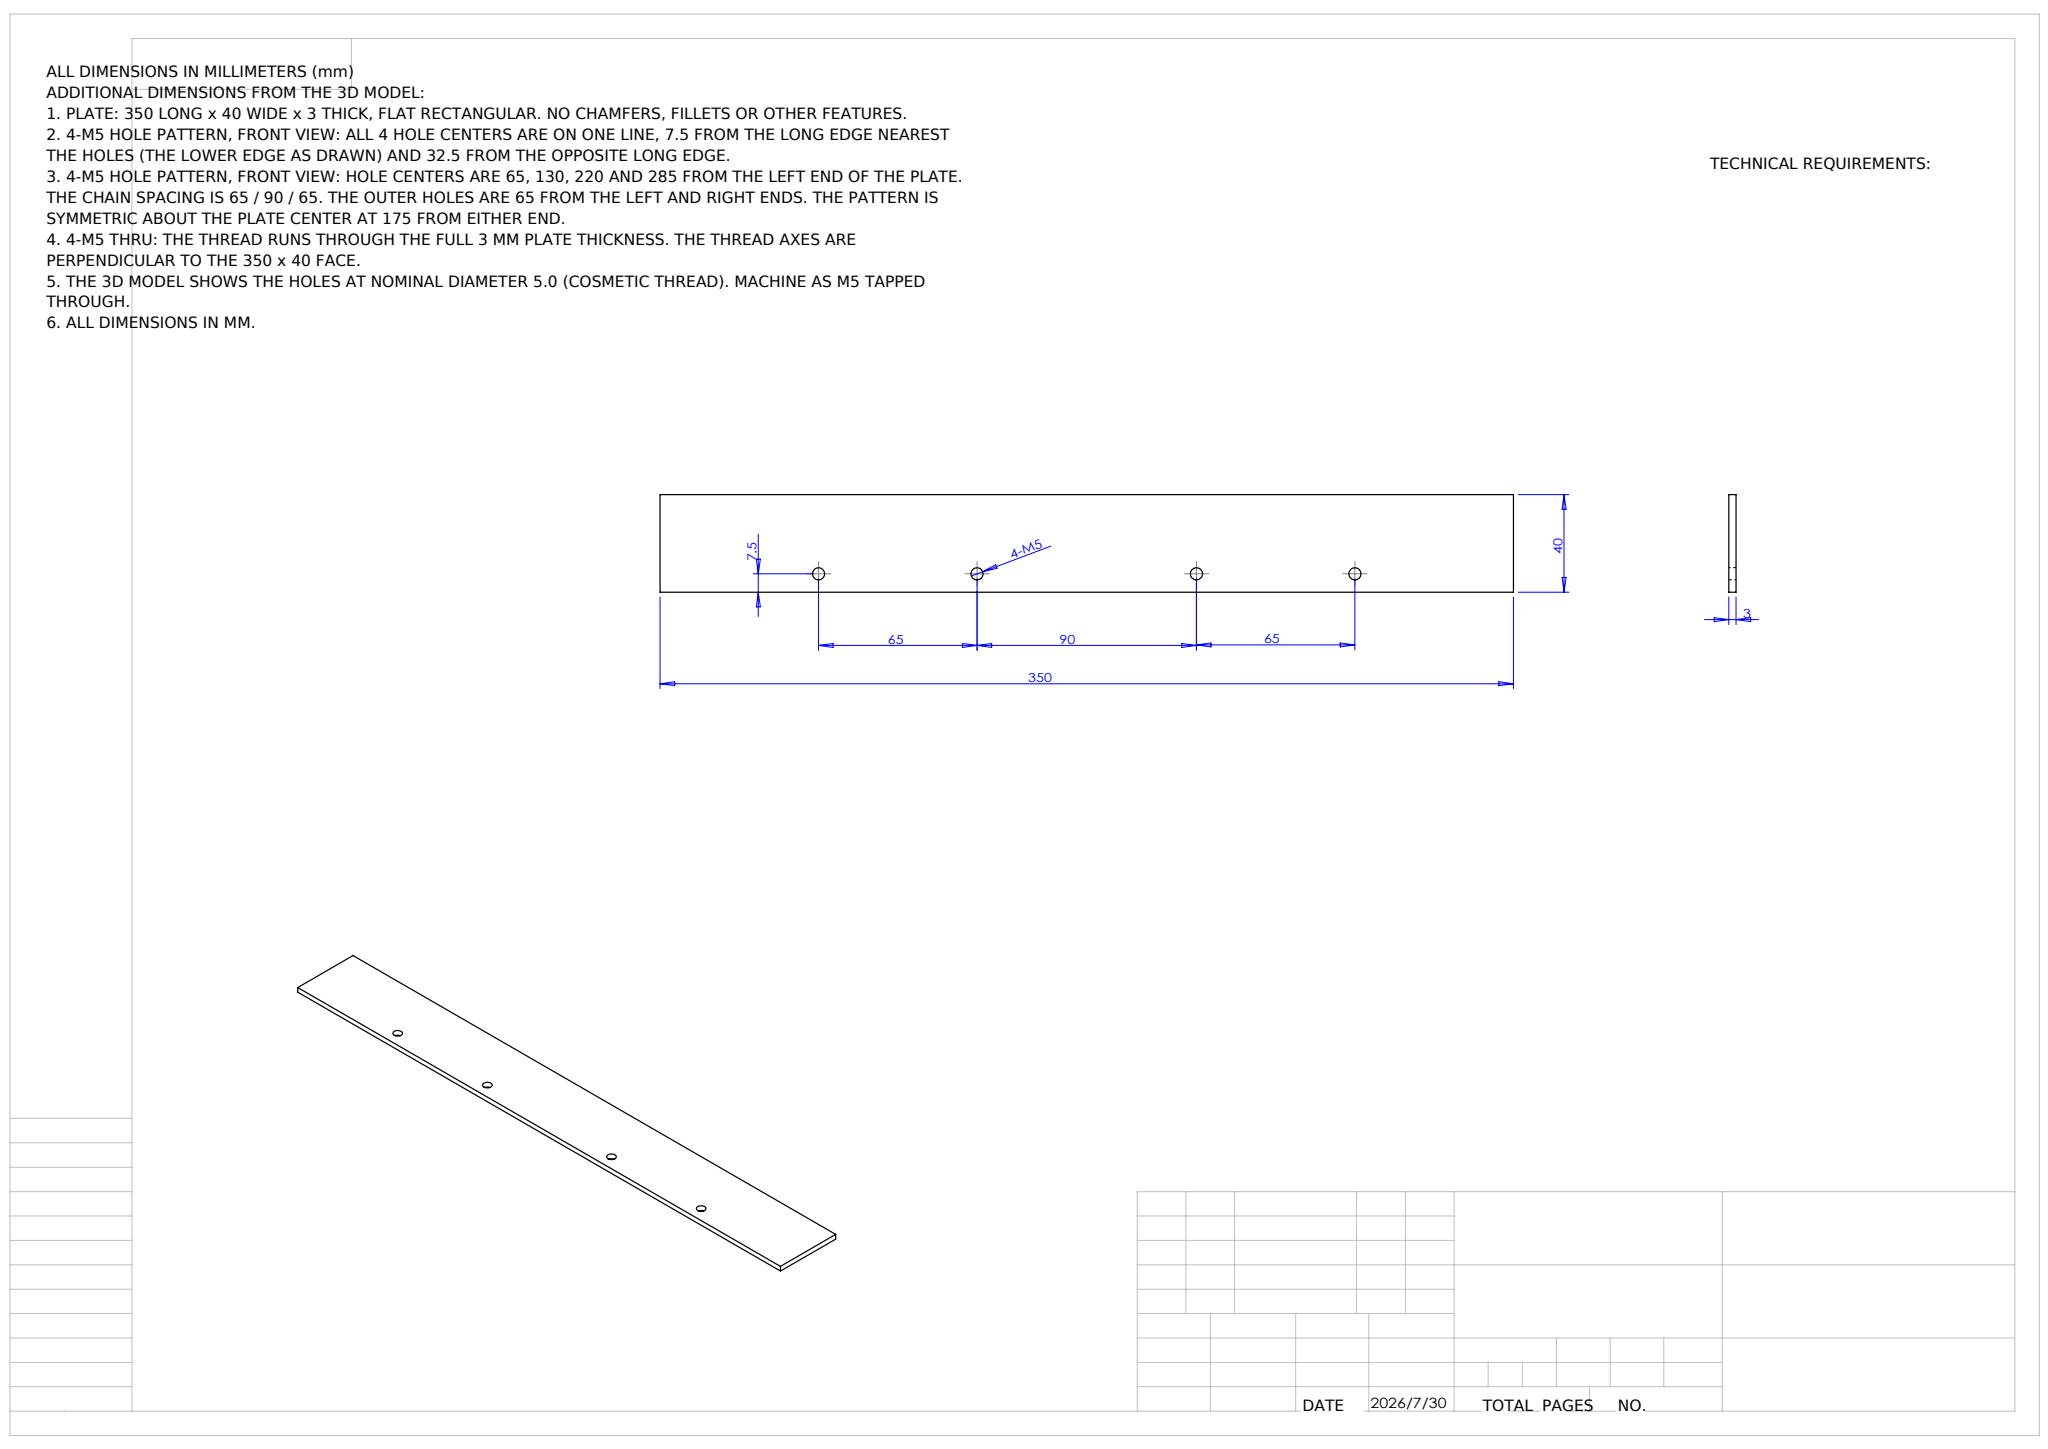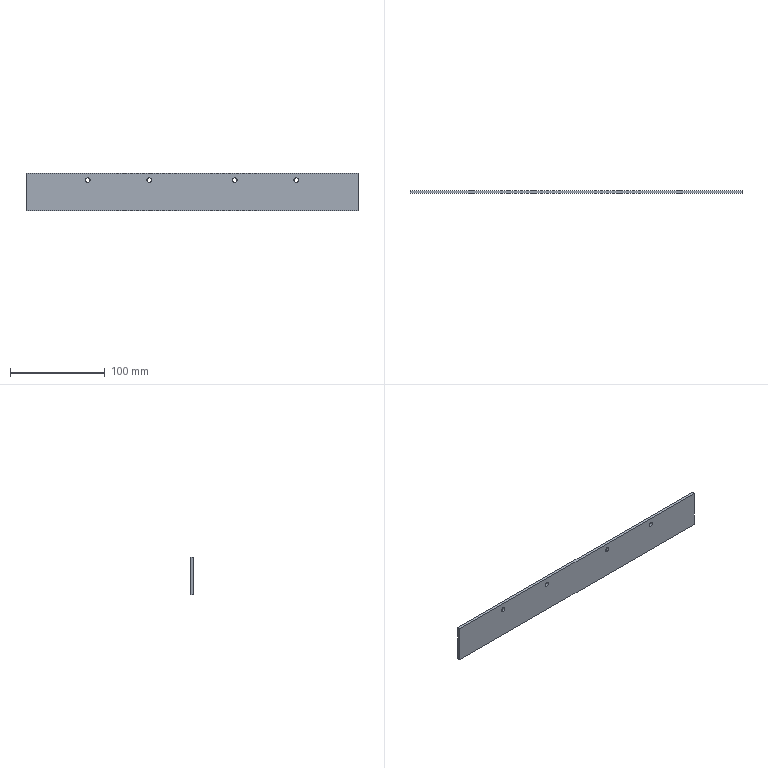Part | NX | mm | 1 solid | 14 faces | box 350 x 3 x 40 mm | volume 41764 mm3 | cylinder 8 | plane 6 | commonest cylinder face diameters 5 x8
STEP:
#1=COLOUR_RGB('',0.7529,0.7529,0.7529);
#2=FILL_AREA_STYLE_COLOUR('',#1);
#3=FILL_AREA_STYLE('',(#2));
#4=SURFACE_STYLE_FILL_AREA(#3);
#5=SURFACE_SIDE_STYLE('',(#4));
#6=SURFACE_STYLE_USAGE(.BOTH.,#5);
#7=PRESENTATION_STYLE_ASSIGNMENT((#6));
#8=CARTESIAN_POINT('',(23.046,0.,5.261));
#9=VERTEX_POINT('',#8);
#10=CARTESIAN_POINT('',(23.046,0.,10.261));
#11=VERTEX_POINT('',#10);
#12=CARTESIAN_POINT('',(23.046,0.,7.761));
#13=DIRECTION('',(0.,1.,0.));
#14=DIRECTION('',(0.,0.,1.));
#15=AXIS2_PLACEMENT_3D('',#12,#13,#14);
#16=CIRCLE('',#15,2.5);
#17=EDGE_CURVE('',#9,#11,#16,.T.);
#18=ORIENTED_EDGE('',*,*,#17,.F.);
#19=CARTESIAN_POINT('',(23.046,3.,5.261));
#20=VERTEX_POINT('',#19);
#21=CARTESIAN_POINT('',(23.046,0.,5.261));
#22=DIRECTION('',(0.,1.,0.));
#23=VECTOR('',#22,1000.);
#24=LINE('',#21,#23);
#25=EDGE_CURVE('',#9,#20,#24,.T.);
#26=ORIENTED_EDGE('',*,*,#25,.T.);
#27=CARTESIAN_POINT('',(23.046,3.,10.261));
#28=VERTEX_POINT('',#27);
#29=CARTESIAN_POINT('',(23.046,3.,7.761));
#30=DIRECTION('',(0.,1.,0.));
#31=DIRECTION('',(0.,0.,1.));
#32=AXIS2_PLACEMENT_3D('',#29,#30,#31);
#33=CIRCLE('',#32,2.5);
#34=EDGE_CURVE('',#20,#28,#33,.T.);
#35=ORIENTED_EDGE('',*,*,#34,.T.);
#36=CARTESIAN_POINT('',(23.046,0.,10.261));
#37=DIRECTION('',(0.,1.,0.));
#38=VECTOR('',#37,1000.);
#39=LINE('',#36,#38);
#40=EDGE_CURVE('',#11,#28,#39,.T.);
#41=ORIENTED_EDGE('',*,*,#40,.F.);
#42=EDGE_LOOP('',(#18,#26,#35,#41));
#43=FACE_OUTER_BOUND('',#42,.T.);
#44=CARTESIAN_POINT('',(23.046,0.,7.761));
#45=DIRECTION('',(0.,1.,0.));
#46=DIRECTION('',(0.,0.,1.));
#47=AXIS2_PLACEMENT_3D('',#44,#45,#46);
#48=CYLINDRICAL_SURFACE('',#47,2.5);
#49=ADVANCED_FACE('',(#43),#48,.F.);
#50=CARTESIAN_POINT('',(-41.954,0.,5.261));
#51=VERTEX_POINT('',#50);
#52=CARTESIAN_POINT('',(-41.954,0.,10.261));
#53=VERTEX_POINT('',#52);
#54=CARTESIAN_POINT('',(-41.954,0.,7.761));
#55=DIRECTION('',(0.,1.,0.));
#56=DIRECTION('',(0.,0.,1.));
#57=AXIS2_PLACEMENT_3D('',#54,#55,#56);
#58=CIRCLE('',#57,2.5);
#59=EDGE_CURVE('',#51,#53,#58,.T.);
#60=ORIENTED_EDGE('',*,*,#59,.F.);
#61=CARTESIAN_POINT('',(-41.954,3.,5.261));
#62=VERTEX_POINT('',#61);
#63=CARTESIAN_POINT('',(-41.954,0.,5.261));
#64=DIRECTION('',(0.,1.,0.));
#65=VECTOR('',#64,1000.);
#66=LINE('',#63,#65);
#67=EDGE_CURVE('',#51,#62,#66,.T.);
#68=ORIENTED_EDGE('',*,*,#67,.T.);
#69=CARTESIAN_POINT('',(-41.954,3.,10.261));
#70=VERTEX_POINT('',#69);
#71=CARTESIAN_POINT('',(-41.954,3.,7.761));
#72=DIRECTION('',(0.,1.,0.));
#73=DIRECTION('',(0.,0.,1.));
#74=AXIS2_PLACEMENT_3D('',#71,#72,#73);
#75=CIRCLE('',#74,2.5);
#76=EDGE_CURVE('',#62,#70,#75,.T.);
#77=ORIENTED_EDGE('',*,*,#76,.T.);
#78=CARTESIAN_POINT('',(-41.954,0.,10.261));
#79=DIRECTION('',(0.,1.,0.));
#80=VECTOR('',#79,1000.);
#81=LINE('',#78,#80);
#82=EDGE_CURVE('',#53,#70,#81,.T.);
#83=ORIENTED_EDGE('',*,*,#82,.F.);
#84=EDGE_LOOP('',(#60,#68,#77,#83));
#85=FACE_OUTER_BOUND('',#84,.T.);
#86=CARTESIAN_POINT('',(-41.954,0.,7.761));
#87=DIRECTION('',(0.,1.,0.));
#88=DIRECTION('',(0.,0.,1.));
#89=AXIS2_PLACEMENT_3D('',#86,#87,#88);
#90=CYLINDRICAL_SURFACE('',#89,2.5);
#91=ADVANCED_FACE('',(#85),#90,.F.);
#92=CARTESIAN_POINT('',(-131.954,0.,5.261));
#93=VERTEX_POINT('',#92);
#94=CARTESIAN_POINT('',(-131.954,0.,10.261));
#95=VERTEX_POINT('',#94);
#96=CARTESIAN_POINT('',(-131.954,0.,7.761));
#97=DIRECTION('',(0.,1.,0.));
#98=DIRECTION('',(0.,0.,1.));
#99=AXIS2_PLACEMENT_3D('',#96,#97,#98);
#100=CIRCLE('',#99,2.5);
#101=EDGE_CURVE('',#93,#95,#100,.T.);
#102=ORIENTED_EDGE('',*,*,#101,.F.);
#103=CARTESIAN_POINT('',(-131.954,3.,5.261));
#104=VERTEX_POINT('',#103);
#105=CARTESIAN_POINT('',(-131.954,0.,5.261));
#106=DIRECTION('',(0.,1.,0.));
#107=VECTOR('',#106,1000.);
#108=LINE('',#105,#107);
#109=EDGE_CURVE('',#93,#104,#108,.T.);
#110=ORIENTED_EDGE('',*,*,#109,.T.);
#111=CARTESIAN_POINT('',(-131.954,3.,10.261));
#112=VERTEX_POINT('',#111);
#113=CARTESIAN_POINT('',(-131.954,3.,7.761));
#114=DIRECTION('',(0.,1.,0.));
#115=DIRECTION('',(0.,0.,1.));
#116=AXIS2_PLACEMENT_3D('',#113,#114,#115);
#117=CIRCLE('',#116,2.5);
#118=EDGE_CURVE('',#104,#112,#117,.T.);
#119=ORIENTED_EDGE('',*,*,#118,.T.);
#120=CARTESIAN_POINT('',(-131.954,0.,10.261));
#121=DIRECTION('',(0.,1.,0.));
#122=VECTOR('',#121,1000.);
#123=LINE('',#120,#122);
#124=EDGE_CURVE('',#95,#112,#123,.T.);
#125=ORIENTED_EDGE('',*,*,#124,.F.);
#126=EDGE_LOOP('',(#102,#110,#119,#125));
#127=FACE_OUTER_BOUND('',#126,.T.);
#128=CARTESIAN_POINT('',(-131.954,0.,7.761));
#129=DIRECTION('',(0.,1.,0.));
#130=DIRECTION('',(0.,0.,1.));
#131=AXIS2_PLACEMENT_3D('',#128,#129,#130);
#132=CYLINDRICAL_SURFACE('',#131,2.5);
#133=ADVANCED_FACE('',(#127),#132,.F.);
#134=CARTESIAN_POINT('',(-196.954,0.,5.261));
#135=VERTEX_POINT('',#134);
#136=CARTESIAN_POINT('',(-196.954,0.,10.261));
#137=VERTEX_POINT('',#136);
#138=CARTESIAN_POINT('',(-196.954,0.,7.761));
#139=DIRECTION('',(0.,1.,0.));
#140=DIRECTION('',(0.,0.,1.));
#141=AXIS2_PLACEMENT_3D('',#138,#139,#140);
#142=CIRCLE('',#141,2.5);
#143=EDGE_CURVE('',#135,#137,#142,.T.);
#144=ORIENTED_EDGE('',*,*,#143,.F.);
#145=CARTESIAN_POINT('',(-196.954,3.,5.261));
#146=VERTEX_POINT('',#145);
#147=CARTESIAN_POINT('',(-196.954,0.,5.261));
#148=DIRECTION('',(0.,1.,0.));
#149=VECTOR('',#148,1000.);
#150=LINE('',#147,#149);
#151=EDGE_CURVE('',#135,#146,#150,.T.);
#152=ORIENTED_EDGE('',*,*,#151,.T.);
#153=CARTESIAN_POINT('',(-196.954,3.,10.261));
#154=VERTEX_POINT('',#153);
#155=CARTESIAN_POINT('',(-196.954,3.,7.761));
#156=DIRECTION('',(0.,1.,0.));
#157=DIRECTION('',(0.,0.,1.));
#158=AXIS2_PLACEMENT_3D('',#155,#156,#157);
#159=CIRCLE('',#158,2.5);
#160=EDGE_CURVE('',#146,#154,#159,.T.);
#161=ORIENTED_EDGE('',*,*,#160,.T.);
#162=CARTESIAN_POINT('',(-196.954,0.,10.261));
#163=DIRECTION('',(0.,1.,0.));
#164=VECTOR('',#163,1000.);
#165=LINE('',#162,#164);
#166=EDGE_CURVE('',#137,#154,#165,.T.);
#167=ORIENTED_EDGE('',*,*,#166,.F.);
#168=EDGE_LOOP('',(#144,#152,#161,#167));
#169=FACE_OUTER_BOUND('',#168,.T.);
#170=CARTESIAN_POINT('',(-196.954,0.,7.761));
#171=DIRECTION('',(0.,1.,0.));
#172=DIRECTION('',(0.,0.,1.));
#173=AXIS2_PLACEMENT_3D('',#170,#171,#172);
#174=CYLINDRICAL_SURFACE('',#173,2.5);
#175=ADVANCED_FACE('',(#169),#174,.F.);
#176=CARTESIAN_POINT('',(-261.954,0.,-24.739));
#177=VERTEX_POINT('',#176);
#178=CARTESIAN_POINT('',(-261.954,0.,15.261));
#179=VERTEX_POINT('',#178);
#180=CARTESIAN_POINT('',(-261.954,0.,15.261));
#181=DIRECTION('',(0.,0.,1.));
#182=VECTOR('',#181,1000.);
#183=LINE('',#180,#182);
#184=EDGE_CURVE('',#177,#179,#183,.T.);
#185=ORIENTED_EDGE('',*,*,#184,.T.);
#186=CARTESIAN_POINT('',(-261.954,3.,15.261));
#187=VERTEX_POINT('',#186);
#188=CARTESIAN_POINT('',(-261.954,3.,15.261));
#189=DIRECTION('',(0.,-1.,0.));
#190=VECTOR('',#189,1000.);
#191=LINE('',#188,#190);
#192=EDGE_CURVE('',#187,#179,#191,.T.);
#193=ORIENTED_EDGE('',*,*,#192,.F.);
#194=CARTESIAN_POINT('',(-261.954,3.,-24.739));
#195=VERTEX_POINT('',#194);
#196=CARTESIAN_POINT('',(-261.954,3.,15.261));
#197=DIRECTION('',(0.,0.,1.));
#198=VECTOR('',#197,1000.);
#199=LINE('',#196,#198);
#200=EDGE_CURVE('',#195,#187,#199,.T.);
#201=ORIENTED_EDGE('',*,*,#200,.F.);
#202=CARTESIAN_POINT('',(-261.954,3.,-24.739));
#203=DIRECTION('',(0.,-1.,0.));
#204=VECTOR('',#203,1000.);
#205=LINE('',#202,#204);
#206=EDGE_CURVE('',#195,#177,#205,.T.);
#207=ORIENTED_EDGE('',*,*,#206,.T.);
#208=EDGE_LOOP('',(#185,#193,#201,#207));
#209=FACE_OUTER_BOUND('',#208,.T.);
#210=CARTESIAN_POINT('',(-261.954,3.,15.261));
#211=DIRECTION('',(1.,0.,0.));
#212=DIRECTION('',(0.,0.,-1.));
#213=AXIS2_PLACEMENT_3D('',#210,#211,#212);
#214=PLANE('',#213);
#215=ADVANCED_FACE('',(#209),#214,.F.);
#216=CARTESIAN_POINT('',(88.046,0.,15.261));
#217=VERTEX_POINT('',#216);
#218=CARTESIAN_POINT('',(-261.954,0.,15.261));
#219=DIRECTION('',(1.,0.,0.));
#220=VECTOR('',#219,1000.);
#221=LINE('',#218,#220);
#222=EDGE_CURVE('',#179,#217,#221,.T.);
#223=ORIENTED_EDGE('',*,*,#222,.T.);
#224=CARTESIAN_POINT('',(88.046,3.,15.261));
#225=VERTEX_POINT('',#224);
#226=CARTESIAN_POINT('',(88.046,3.,15.261));
#227=DIRECTION('',(0.,-1.,0.));
#228=VECTOR('',#227,1000.);
#229=LINE('',#226,#228);
#230=EDGE_CURVE('',#225,#217,#229,.T.);
#231=ORIENTED_EDGE('',*,*,#230,.F.);
#232=CARTESIAN_POINT('',(-261.954,3.,15.261));
#233=DIRECTION('',(1.,0.,0.));
#234=VECTOR('',#233,1000.);
#235=LINE('',#232,#234);
#236=EDGE_CURVE('',#187,#225,#235,.T.);
#237=ORIENTED_EDGE('',*,*,#236,.F.);
#238=ORIENTED_EDGE('',*,*,#192,.T.);
#239=EDGE_LOOP('',(#223,#231,#237,#238));
#240=FACE_OUTER_BOUND('',#239,.T.);
#241=CARTESIAN_POINT('',(-261.954,3.,15.261));
#242=DIRECTION('',(0.,0.,-1.));
#243=DIRECTION('',(-1.,0.,0.));
#244=AXIS2_PLACEMENT_3D('',#241,#242,#243);
#245=PLANE('',#244);
#246=ADVANCED_FACE('',(#240),#245,.F.);
#247=CARTESIAN_POINT('',(88.046,0.,-24.739));
#248=VERTEX_POINT('',#247);
#249=CARTESIAN_POINT('',(88.046,0.,15.261));
#250=DIRECTION('',(0.,0.,-1.));
#251=VECTOR('',#250,1000.);
#252=LINE('',#249,#251);
#253=EDGE_CURVE('',#217,#248,#252,.T.);
#254=ORIENTED_EDGE('',*,*,#253,.T.);
#255=CARTESIAN_POINT('',(88.046,3.,-24.739));
#256=VERTEX_POINT('',#255);
#257=CARTESIAN_POINT('',(88.046,3.,-24.739));
#258=DIRECTION('',(0.,-1.,0.));
#259=VECTOR('',#258,1000.);
#260=LINE('',#257,#259);
#261=EDGE_CURVE('',#256,#248,#260,.T.);
#262=ORIENTED_EDGE('',*,*,#261,.F.);
#263=CARTESIAN_POINT('',(88.046,3.,15.261));
#264=DIRECTION('',(0.,0.,-1.));
#265=VECTOR('',#264,1000.);
#266=LINE('',#263,#265);
#267=EDGE_CURVE('',#225,#256,#266,.T.);
#268=ORIENTED_EDGE('',*,*,#267,.F.);
#269=ORIENTED_EDGE('',*,*,#230,.T.);
#270=EDGE_LOOP('',(#254,#262,#268,#269));
#271=FACE_OUTER_BOUND('',#270,.T.);
#272=CARTESIAN_POINT('',(88.046,3.,15.261));
#273=DIRECTION('',(-1.,0.,0.));
#274=DIRECTION('',(0.,0.,1.));
#275=AXIS2_PLACEMENT_3D('',#272,#273,#274);
#276=PLANE('',#275);
#277=ADVANCED_FACE('',(#271),#276,.F.);
#278=CARTESIAN_POINT('',(-261.954,0.,-24.739));
#279=DIRECTION('',(-1.,0.,0.));
#280=VECTOR('',#279,1000.);
#281=LINE('',#278,#280);
#282=EDGE_CURVE('',#248,#177,#281,.T.);
#283=ORIENTED_EDGE('',*,*,#282,.T.);
#284=ORIENTED_EDGE('',*,*,#206,.F.);
#285=CARTESIAN_POINT('',(-261.954,3.,-24.739));
#286=DIRECTION('',(-1.,0.,0.));
#287=VECTOR('',#286,1000.);
#288=LINE('',#285,#287);
#289=EDGE_CURVE('',#256,#195,#288,.T.);
#290=ORIENTED_EDGE('',*,*,#289,.F.);
#291=ORIENTED_EDGE('',*,*,#261,.T.);
#292=EDGE_LOOP('',(#283,#284,#290,#291));
#293=FACE_OUTER_BOUND('',#292,.T.);
#294=CARTESIAN_POINT('',(-261.954,3.,-24.739));
#295=DIRECTION('',(0.,0.,1.));
#296=DIRECTION('',(1.,0.,0.));
#297=AXIS2_PLACEMENT_3D('',#294,#295,#296);
#298=PLANE('',#297);
#299=ADVANCED_FACE('',(#293),#298,.F.);
#300=CARTESIAN_POINT('',(23.046,3.,7.761));
#301=DIRECTION('',(0.,1.,0.));
#302=DIRECTION('',(0.,0.,1.));
#303=AXIS2_PLACEMENT_3D('',#300,#301,#302);
#304=CIRCLE('',#303,2.5);
#305=EDGE_CURVE('',#28,#20,#304,.T.);
#306=ORIENTED_EDGE('',*,*,#305,.F.);
#307=ORIENTED_EDGE('',*,*,#34,.F.);
#308=EDGE_LOOP('',(#306,#307));
#309=FACE_BOUND('',#308,.T.);
#310=CARTESIAN_POINT('',(-41.954,3.,7.761));
#311=DIRECTION('',(0.,1.,0.));
#312=DIRECTION('',(0.,0.,1.));
#313=AXIS2_PLACEMENT_3D('',#310,#311,#312);
#314=CIRCLE('',#313,2.5);
#315=EDGE_CURVE('',#70,#62,#314,.T.);
#316=ORIENTED_EDGE('',*,*,#315,.F.);
#317=ORIENTED_EDGE('',*,*,#76,.F.);
#318=EDGE_LOOP('',(#316,#317));
#319=FACE_BOUND('',#318,.T.);
#320=CARTESIAN_POINT('',(-131.954,3.,7.761));
#321=DIRECTION('',(0.,1.,0.));
#322=DIRECTION('',(0.,0.,1.));
#323=AXIS2_PLACEMENT_3D('',#320,#321,#322);
#324=CIRCLE('',#323,2.5);
#325=EDGE_CURVE('',#112,#104,#324,.T.);
#326=ORIENTED_EDGE('',*,*,#325,.F.);
#327=ORIENTED_EDGE('',*,*,#118,.F.);
#328=EDGE_LOOP('',(#326,#327));
#329=FACE_BOUND('',#328,.T.);
#330=CARTESIAN_POINT('',(-196.954,3.,7.761));
#331=DIRECTION('',(0.,1.,0.));
#332=DIRECTION('',(0.,0.,1.));
#333=AXIS2_PLACEMENT_3D('',#330,#331,#332);
#334=CIRCLE('',#333,2.5);
#335=EDGE_CURVE('',#154,#146,#334,.T.);
#336=ORIENTED_EDGE('',*,*,#335,.F.);
#337=ORIENTED_EDGE('',*,*,#160,.F.);
#338=EDGE_LOOP('',(#336,#337));
#339=FACE_BOUND('',#338,.T.);
#340=ORIENTED_EDGE('',*,*,#200,.T.);
#341=ORIENTED_EDGE('',*,*,#236,.T.);
#342=ORIENTED_EDGE('',*,*,#267,.T.);
#343=ORIENTED_EDGE('',*,*,#289,.T.);
#344=EDGE_LOOP('',(#340,#341,#342,#343));
#345=FACE_OUTER_BOUND('',#344,.T.);
#346=CARTESIAN_POINT('',(-261.954,3.,-24.739));
#347=DIRECTION('',(0.,-1.,0.));
#348=DIRECTION('',(0.,0.,-1.));
#349=AXIS2_PLACEMENT_3D('',#346,#347,#348);
#350=PLANE('',#349);
#351=ADVANCED_FACE('',(#309,#319,#329,#339,#345),#350,.F.);
#352=CARTESIAN_POINT('',(23.046,0.,7.761));
#353=DIRECTION('',(0.,1.,0.));
#354=DIRECTION('',(0.,0.,1.));
#355=AXIS2_PLACEMENT_3D('',#352,#353,#354);
#356=CIRCLE('',#355,2.5);
#357=EDGE_CURVE('',#11,#9,#356,.T.);
#358=ORIENTED_EDGE('',*,*,#357,.T.);
#359=ORIENTED_EDGE('',*,*,#17,.T.);
#360=EDGE_LOOP('',(#358,#359));
#361=FACE_BOUND('',#360,.T.);
#362=CARTESIAN_POINT('',(-41.954,0.,7.761));
#363=DIRECTION('',(0.,1.,0.));
#364=DIRECTION('',(0.,0.,1.));
#365=AXIS2_PLACEMENT_3D('',#362,#363,#364);
#366=CIRCLE('',#365,2.5);
#367=EDGE_CURVE('',#53,#51,#366,.T.);
#368=ORIENTED_EDGE('',*,*,#367,.T.);
#369=ORIENTED_EDGE('',*,*,#59,.T.);
#370=EDGE_LOOP('',(#368,#369));
#371=FACE_BOUND('',#370,.T.);
#372=CARTESIAN_POINT('',(-131.954,0.,7.761));
#373=DIRECTION('',(0.,1.,0.));
#374=DIRECTION('',(0.,0.,1.));
#375=AXIS2_PLACEMENT_3D('',#372,#373,#374);
#376=CIRCLE('',#375,2.5);
#377=EDGE_CURVE('',#95,#93,#376,.T.);
#378=ORIENTED_EDGE('',*,*,#377,.T.);
#379=ORIENTED_EDGE('',*,*,#101,.T.);
#380=EDGE_LOOP('',(#378,#379));
#381=FACE_BOUND('',#380,.T.);
#382=CARTESIAN_POINT('',(-196.954,0.,7.761));
#383=DIRECTION('',(0.,1.,0.));
#384=DIRECTION('',(0.,0.,1.));
#385=AXIS2_PLACEMENT_3D('',#382,#383,#384);
#386=CIRCLE('',#385,2.5);
#387=EDGE_CURVE('',#137,#135,#386,.T.);
#388=ORIENTED_EDGE('',*,*,#387,.T.);
#389=ORIENTED_EDGE('',*,*,#143,.T.);
#390=EDGE_LOOP('',(#388,#389));
#391=FACE_BOUND('',#390,.T.);
#392=ORIENTED_EDGE('',*,*,#184,.F.);
#393=ORIENTED_EDGE('',*,*,#282,.F.);
#394=ORIENTED_EDGE('',*,*,#253,.F.);
#395=ORIENTED_EDGE('',*,*,#222,.F.);
#396=EDGE_LOOP('',(#392,#393,#394,#395));
#397=FACE_OUTER_BOUND('',#396,.T.);
#398=CARTESIAN_POINT('',(-261.954,0.,-24.739));
#399=DIRECTION('',(0.,-1.,0.));
#400=DIRECTION('',(0.,0.,-1.));
#401=AXIS2_PLACEMENT_3D('',#398,#399,#400);
#402=PLANE('',#401);
#403=ADVANCED_FACE('',(#361,#371,#381,#391,#397),#402,.T.);
#404=ORIENTED_EDGE('',*,*,#151,.F.);
#405=ORIENTED_EDGE('',*,*,#387,.F.);
#406=ORIENTED_EDGE('',*,*,#166,.T.);
#407=ORIENTED_EDGE('',*,*,#335,.T.);
#408=EDGE_LOOP('',(#404,#405,#406,#407));
#409=FACE_OUTER_BOUND('',#408,.T.);
#410=CARTESIAN_POINT('',(-196.954,0.,7.761));
#411=DIRECTION('',(0.,1.,0.));
#412=DIRECTION('',(0.,0.,1.));
#413=AXIS2_PLACEMENT_3D('',#410,#411,#412);
#414=CYLINDRICAL_SURFACE('',#413,2.5);
#415=ADVANCED_FACE('',(#409),#414,.F.);
#416=ORIENTED_EDGE('',*,*,#109,.F.);
#417=ORIENTED_EDGE('',*,*,#377,.F.);
#418=ORIENTED_EDGE('',*,*,#124,.T.);
#419=ORIENTED_EDGE('',*,*,#325,.T.);
#420=EDGE_LOOP('',(#416,#417,#418,#419));
#421=FACE_OUTER_BOUND('',#420,.T.);
#422=CARTESIAN_POINT('',(-131.954,0.,7.761));
#423=DIRECTION('',(0.,1.,0.));
#424=DIRECTION('',(0.,0.,1.));
#425=AXIS2_PLACEMENT_3D('',#422,#423,#424);
#426=CYLINDRICAL_SURFACE('',#425,2.5);
#427=ADVANCED_FACE('',(#421),#426,.F.);
#428=ORIENTED_EDGE('',*,*,#67,.F.);
#429=ORIENTED_EDGE('',*,*,#367,.F.);
#430=ORIENTED_EDGE('',*,*,#82,.T.);
#431=ORIENTED_EDGE('',*,*,#315,.T.);
#432=EDGE_LOOP('',(#428,#429,#430,#431));
#433=FACE_OUTER_BOUND('',#432,.T.);
#434=CARTESIAN_POINT('',(-41.954,0.,7.761));
#435=DIRECTION('',(0.,1.,0.));
#436=DIRECTION('',(0.,0.,1.));
#437=AXIS2_PLACEMENT_3D('',#434,#435,#436);
#438=CYLINDRICAL_SURFACE('',#437,2.5);
#439=ADVANCED_FACE('',(#433),#438,.F.);
#440=ORIENTED_EDGE('',*,*,#25,.F.);
#441=ORIENTED_EDGE('',*,*,#357,.F.);
#442=ORIENTED_EDGE('',*,*,#40,.T.);
#443=ORIENTED_EDGE('',*,*,#305,.T.);
#444=EDGE_LOOP('',(#440,#441,#442,#443));
#445=FACE_OUTER_BOUND('',#444,.T.);
#446=CARTESIAN_POINT('',(23.046,0.,7.761));
#447=DIRECTION('',(0.,1.,0.));
#448=DIRECTION('',(0.,0.,1.));
#449=AXIS2_PLACEMENT_3D('',#446,#447,#448);
#450=CYLINDRICAL_SURFACE('',#449,2.5);
#451=ADVANCED_FACE('',(#445),#450,.F.);
#452=CLOSED_SHELL('',(#49,#91,#133,#175,#215,#246,#277,#299,#351,#403,#415,#427,#439,#451));
#453=MANIFOLD_SOLID_BREP('',#452);
#454=STYLED_ITEM('',(#7),#453);
#455=(LENGTH_UNIT()NAMED_UNIT(*)SI_UNIT(.MILLI.,.METRE.));
#456=UNCERTAINTY_MEASURE_WITH_UNIT(LENGTH_MEASURE(0.00001),#455,'','');
#457=(NAMED_UNIT(*)PLANE_ANGLE_UNIT()SI_UNIT($,.RADIAN.));
#458=(NAMED_UNIT(*)SI_UNIT($,.STERADIAN.)SOLID_ANGLE_UNIT());
#459=(GEOMETRIC_REPRESENTATION_CONTEXT(3)GLOBAL_UNCERTAINTY_ASSIGNED_CONTEXT((#456))GLOBAL_UNIT_ASSIGNED_CONTEXT((#455,#457,#458))REPRESENTATION_CONTEXT('',''));
#460=MECHANICAL_DESIGN_GEOMETRIC_PRESENTATION_REPRESENTATION('',(#454),#459);
#461=COLOUR_RGB('',0.7529,0.7529,0.7529);
#462=FILL_AREA_STYLE_COLOUR('',#461);
#463=FILL_AREA_STYLE('',(#462));
#464=SURFACE_STYLE_FILL_AREA(#463);
#465=SURFACE_SIDE_STYLE('',(#464));
#466=SURFACE_STYLE_USAGE(.BOTH.,#465);
#467=PRESENTATION_STYLE_ASSIGNMENT((#466));
#468=CARTESIAN_POINT('',(0.,0.,0.));
#469=DIRECTION('',(0.,0.,1.));
#470=DIRECTION('',(1.,0.,0.));
#471=AXIS2_PLACEMENT_3D('',#468,#469,#470);
#472=(LENGTH_UNIT()NAMED_UNIT(*)SI_UNIT(.MILLI.,.METRE.));
#473=UNCERTAINTY_MEASURE_WITH_UNIT(LENGTH_MEASURE(0.00001),#472,'','');
#474=(NAMED_UNIT(*)PLANE_ANGLE_UNIT()SI_UNIT($,.RADIAN.));
#475=(NAMED_UNIT(*)SI_UNIT($,.STERADIAN.)SOLID_ANGLE_UNIT());
#476=(GEOMETRIC_REPRESENTATION_CONTEXT(3)GLOBAL_UNCERTAINTY_ASSIGNED_CONTEXT((#473))GLOBAL_UNIT_ASSIGNED_CONTEXT((#472,#474,#475))REPRESENTATION_CONTEXT('',''));
#477=ADVANCED_BREP_SHAPE_REPRESENTATION('',(#453,#471),#476);
#478=STYLED_ITEM('',(#467),#477);
#479=(LENGTH_UNIT()NAMED_UNIT(*)SI_UNIT(.MILLI.,.METRE.));
#480=UNCERTAINTY_MEASURE_WITH_UNIT(LENGTH_MEASURE(0.00001),#479,'','');
#481=(NAMED_UNIT(*)PLANE_ANGLE_UNIT()SI_UNIT($,.RADIAN.));
#482=(NAMED_UNIT(*)SI_UNIT($,.STERADIAN.)SOLID_ANGLE_UNIT());
#483=(GEOMETRIC_REPRESENTATION_CONTEXT(3)GLOBAL_UNCERTAINTY_ASSIGNED_CONTEXT((#480))GLOBAL_UNIT_ASSIGNED_CONTEXT((#479,#481,#482))REPRESENTATION_CONTEXT('',''));
#484=MECHANICAL_DESIGN_GEOMETRIC_PRESENTATION_REPRESENTATION('',(#478),#483);
#485=PRESENTATION_LAYER_ASSIGNMENT('','',(#454));
#486=PRESENTATION_LAYER_ASSIGNMENT('','',(#478));